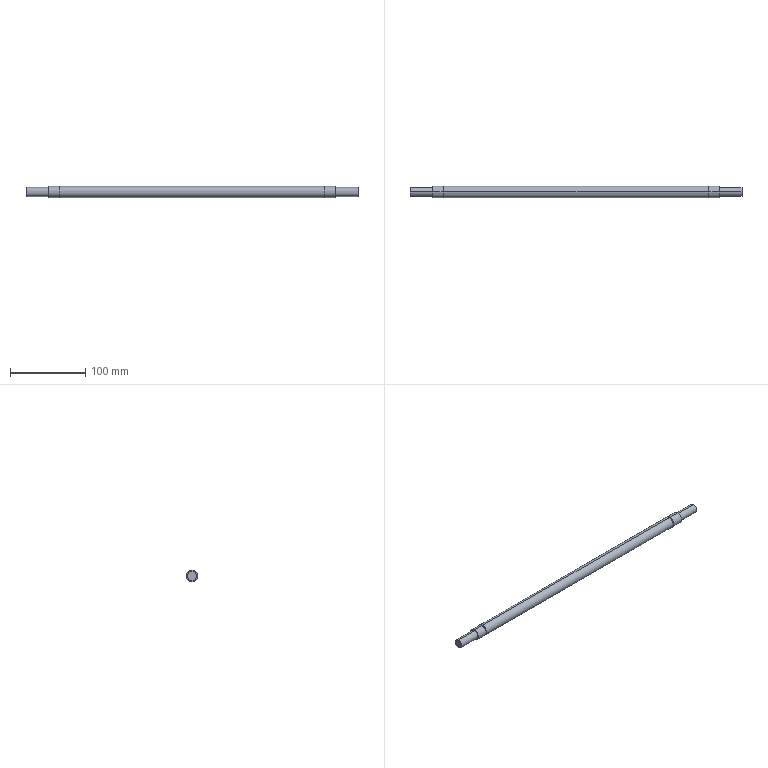Component | SolidWorks | 01-09MarkingMachineIdlerRollerAxis-2 | 1 solid | 22 faces | box 440 x 15 x 15 mm | volume 73902 mm3 | cylinder 14 | plane 8 | commonest cylinder face diameters 15 x6 12 x4 14.3 x4 | material A3 Steel
build123d program:
from build123d import *


with BuildPart() as part:
    # Sketch1 → Revolve1 (revolve)
    with BuildSketch(Plane.XY, mode=Mode.PRIVATE) as revolve1_sk:
        Polygon((-220, 0), (-220, 6), (-190, 6), (-190, 7.5), (-176.1, 7.5), (-176.1, 7.15), (-175, 7.15), (-175, 7.5), (175, 7.5), (175, 7.15), (176.1, 7.15), (176.1, 7.5), (190, 7.5), (190, 6), (220, 6), (220, 0), align=None)
    revolve(revolve1_sk.sketch.rotate(Axis((-253.202, 0, 0), (1, 0, 0)), 90), axis=Axis((-253.202, 0, 0), (1, 0, 0)))


solid = part.part

# Placed as in the assembly
solid = solid.moved(Location((-256.91, 57.41, 27.5), (0, 0, 0)))
STEP:
#1=COLOUR_RGB('',0.7922,0.8196,0.9333);
#2=FILL_AREA_STYLE_COLOUR('',#1);
#3=FILL_AREA_STYLE('',(#2));
#4=SURFACE_STYLE_FILL_AREA(#3);
#5=SURFACE_SIDE_STYLE('',(#4));
#6=SURFACE_STYLE_USAGE(.BOTH.,#5);
#7=PRESENTATION_STYLE_ASSIGNMENT((#6));
#8=CARTESIAN_POINT('',(-17.595,2.26,1.319));
#9=VERTEX_POINT('',#8);
#10=CARTESIAN_POINT('',(-17.595,2.26,0.8465));
#11=VERTEX_POINT('',#10);
#12=CARTESIAN_POINT('',(-17.595,2.26,1.083));
#13=DIRECTION('',(-1.,0.,0.));
#14=DIRECTION('',(0.,0.,1.));
#15=AXIS2_PLACEMENT_3D('',#12,#13,#14);
#16=CIRCLE('',#15,0.2362);
#17=EDGE_CURVE('',#9,#11,#16,.T.);
#18=ORIENTED_EDGE('',*,*,#17,.T.);
#19=CARTESIAN_POINT('',(-18.776,2.26,0.8465));
#20=VERTEX_POINT('',#19);
#21=CARTESIAN_POINT('',(-20.083,2.26,0.8465));
#22=DIRECTION('',(-1.,0.,0.));
#23=VECTOR('',#22,39.37);
#24=LINE('',#21,#23);
#25=EDGE_CURVE('',#11,#20,#24,.T.);
#26=ORIENTED_EDGE('',*,*,#25,.T.);
#27=CARTESIAN_POINT('',(-18.776,2.26,1.319));
#28=VERTEX_POINT('',#27);
#29=CARTESIAN_POINT('',(-18.776,2.26,1.083));
#30=DIRECTION('',(-1.,0.,0.));
#31=DIRECTION('',(0.,0.,1.));
#32=AXIS2_PLACEMENT_3D('',#29,#30,#31);
#33=CIRCLE('',#32,0.2362);
#34=EDGE_CURVE('',#28,#20,#33,.T.);
#35=ORIENTED_EDGE('',*,*,#34,.F.);
#36=CARTESIAN_POINT('',(-20.083,2.26,1.319));
#37=DIRECTION('',(-1.,0.,0.));
#38=VECTOR('',#37,39.37);
#39=LINE('',#36,#38);
#40=EDGE_CURVE('',#9,#28,#39,.T.);
#41=ORIENTED_EDGE('',*,*,#40,.F.);
#42=EDGE_LOOP('',(#18,#26,#35,#41));
#43=FACE_OUTER_BOUND('',#42,.T.);
#44=CARTESIAN_POINT('',(-20.083,2.26,1.083));
#45=DIRECTION('',(-1.,0.,0.));
#46=DIRECTION('',(0.,0.,1.));
#47=AXIS2_PLACEMENT_3D('',#44,#45,#46);
#48=CYLINDRICAL_SURFACE('',#47,0.2362);
#49=ADVANCED_FACE('',(#43),#48,.T.);
#50=CARTESIAN_POINT('',(-17.048,2.26,1.378));
#51=VERTEX_POINT('',#50);
#52=CARTESIAN_POINT('',(-17.048,2.26,0.7874));
#53=VERTEX_POINT('',#52);
#54=CARTESIAN_POINT('',(-17.048,2.26,1.083));
#55=DIRECTION('',(-1.,0.,0.));
#56=DIRECTION('',(0.,0.,1.));
#57=AXIS2_PLACEMENT_3D('',#54,#55,#56);
#58=CIRCLE('',#57,0.2953);
#59=EDGE_CURVE('',#51,#53,#58,.T.);
#60=ORIENTED_EDGE('',*,*,#59,.T.);
#61=CARTESIAN_POINT('',(-17.595,2.26,0.7874));
#62=VERTEX_POINT('',#61);
#63=CARTESIAN_POINT('',(-20.083,2.26,0.7874));
#64=DIRECTION('',(-1.,0.,0.));
#65=VECTOR('',#64,39.37);
#66=LINE('',#63,#65);
#67=EDGE_CURVE('',#53,#62,#66,.T.);
#68=ORIENTED_EDGE('',*,*,#67,.T.);
#69=CARTESIAN_POINT('',(-17.595,2.26,1.378));
#70=VERTEX_POINT('',#69);
#71=CARTESIAN_POINT('',(-17.595,2.26,1.083));
#72=DIRECTION('',(-1.,0.,0.));
#73=DIRECTION('',(0.,0.,1.));
#74=AXIS2_PLACEMENT_3D('',#71,#72,#73);
#75=CIRCLE('',#74,0.2953);
#76=EDGE_CURVE('',#70,#62,#75,.T.);
#77=ORIENTED_EDGE('',*,*,#76,.F.);
#78=CARTESIAN_POINT('',(-20.083,2.26,1.378));
#79=DIRECTION('',(-1.,0.,0.));
#80=VECTOR('',#79,39.37);
#81=LINE('',#78,#80);
#82=EDGE_CURVE('',#51,#70,#81,.T.);
#83=ORIENTED_EDGE('',*,*,#82,.F.);
#84=EDGE_LOOP('',(#60,#68,#77,#83));
#85=FACE_OUTER_BOUND('',#84,.T.);
#86=CARTESIAN_POINT('',(-20.083,2.26,1.083));
#87=DIRECTION('',(-1.,0.,0.));
#88=DIRECTION('',(0.,0.,1.));
#89=AXIS2_PLACEMENT_3D('',#86,#87,#88);
#90=CYLINDRICAL_SURFACE('',#89,0.2953);
#91=ADVANCED_FACE('',(#85),#90,.T.);
#92=CARTESIAN_POINT('',(-17.004,2.26,1.364));
#93=VERTEX_POINT('',#92);
#94=CARTESIAN_POINT('',(-17.004,2.26,0.8012));
#95=VERTEX_POINT('',#94);
#96=CARTESIAN_POINT('',(-17.004,2.26,1.083));
#97=DIRECTION('',(-1.,0.,0.));
#98=DIRECTION('',(0.,0.,1.));
#99=AXIS2_PLACEMENT_3D('',#96,#97,#98);
#100=CIRCLE('',#99,0.2815);
#101=EDGE_CURVE('',#93,#95,#100,.T.);
#102=ORIENTED_EDGE('',*,*,#101,.T.);
#103=CARTESIAN_POINT('',(-17.048,2.26,0.8012));
#104=VERTEX_POINT('',#103);
#105=CARTESIAN_POINT('',(-20.083,2.26,0.8012));
#106=DIRECTION('',(-1.,0.,0.));
#107=VECTOR('',#106,39.37);
#108=LINE('',#105,#107);
#109=EDGE_CURVE('',#95,#104,#108,.T.);
#110=ORIENTED_EDGE('',*,*,#109,.T.);
#111=CARTESIAN_POINT('',(-17.048,2.26,1.364));
#112=VERTEX_POINT('',#111);
#113=CARTESIAN_POINT('',(-17.048,2.26,1.083));
#114=DIRECTION('',(-1.,0.,0.));
#115=DIRECTION('',(0.,0.,1.));
#116=AXIS2_PLACEMENT_3D('',#113,#114,#115);
#117=CIRCLE('',#116,0.2815);
#118=EDGE_CURVE('',#112,#104,#117,.T.);
#119=ORIENTED_EDGE('',*,*,#118,.F.);
#120=CARTESIAN_POINT('',(-20.083,2.26,1.364));
#121=DIRECTION('',(-1.,0.,0.));
#122=VECTOR('',#121,39.37);
#123=LINE('',#120,#122);
#124=EDGE_CURVE('',#93,#112,#123,.T.);
#125=ORIENTED_EDGE('',*,*,#124,.F.);
#126=EDGE_LOOP('',(#102,#110,#119,#125));
#127=FACE_OUTER_BOUND('',#126,.T.);
#128=CARTESIAN_POINT('',(-20.083,2.26,1.083));
#129=DIRECTION('',(-1.,0.,0.));
#130=DIRECTION('',(0.,0.,1.));
#131=AXIS2_PLACEMENT_3D('',#128,#129,#130);
#132=CYLINDRICAL_SURFACE('',#131,0.2815);
#133=ADVANCED_FACE('',(#127),#132,.T.);
#134=CARTESIAN_POINT('',(-3.225,2.26,1.378));
#135=VERTEX_POINT('',#134);
#136=CARTESIAN_POINT('',(-3.225,2.26,0.7874));
#137=VERTEX_POINT('',#136);
#138=CARTESIAN_POINT('',(-3.225,2.26,1.083));
#139=DIRECTION('',(-1.,0.,0.));
#140=DIRECTION('',(0.,0.,1.));
#141=AXIS2_PLACEMENT_3D('',#138,#139,#140);
#142=CIRCLE('',#141,0.2953);
#143=EDGE_CURVE('',#135,#137,#142,.T.);
#144=ORIENTED_EDGE('',*,*,#143,.T.);
#145=CARTESIAN_POINT('',(-17.004,2.26,0.7874));
#146=VERTEX_POINT('',#145);
#147=CARTESIAN_POINT('',(-20.083,2.26,0.7874));
#148=DIRECTION('',(-1.,0.,0.));
#149=VECTOR('',#148,39.37);
#150=LINE('',#147,#149);
#151=EDGE_CURVE('',#137,#146,#150,.T.);
#152=ORIENTED_EDGE('',*,*,#151,.T.);
#153=CARTESIAN_POINT('',(-17.004,2.26,1.378));
#154=VERTEX_POINT('',#153);
#155=CARTESIAN_POINT('',(-17.004,2.26,1.083));
#156=DIRECTION('',(-1.,0.,0.));
#157=DIRECTION('',(0.,0.,1.));
#158=AXIS2_PLACEMENT_3D('',#155,#156,#157);
#159=CIRCLE('',#158,0.2953);
#160=EDGE_CURVE('',#154,#146,#159,.T.);
#161=ORIENTED_EDGE('',*,*,#160,.F.);
#162=CARTESIAN_POINT('',(-20.083,2.26,1.378));
#163=DIRECTION('',(-1.,0.,0.));
#164=VECTOR('',#163,39.37);
#165=LINE('',#162,#164);
#166=EDGE_CURVE('',#135,#154,#165,.T.);
#167=ORIENTED_EDGE('',*,*,#166,.F.);
#168=EDGE_LOOP('',(#144,#152,#161,#167));
#169=FACE_OUTER_BOUND('',#168,.T.);
#170=CARTESIAN_POINT('',(-20.083,2.26,1.083));
#171=DIRECTION('',(-1.,0.,0.));
#172=DIRECTION('',(0.,0.,1.));
#173=AXIS2_PLACEMENT_3D('',#170,#171,#172);
#174=CYLINDRICAL_SURFACE('',#173,0.2953);
#175=ADVANCED_FACE('',(#169),#174,.T.);
#176=CARTESIAN_POINT('',(-3.182,2.26,1.364));
#177=VERTEX_POINT('',#176);
#178=CARTESIAN_POINT('',(-3.182,2.26,0.8012));
#179=VERTEX_POINT('',#178);
#180=CARTESIAN_POINT('',(-3.182,2.26,1.083));
#181=DIRECTION('',(-1.,0.,0.));
#182=DIRECTION('',(0.,0.,1.));
#183=AXIS2_PLACEMENT_3D('',#180,#181,#182);
#184=CIRCLE('',#183,0.2815);
#185=EDGE_CURVE('',#177,#179,#184,.T.);
#186=ORIENTED_EDGE('',*,*,#185,.T.);
#187=CARTESIAN_POINT('',(-3.225,2.26,0.8012));
#188=VERTEX_POINT('',#187);
#189=CARTESIAN_POINT('',(-20.083,2.26,0.8012));
#190=DIRECTION('',(-1.,0.,0.));
#191=VECTOR('',#190,39.37);
#192=LINE('',#189,#191);
#193=EDGE_CURVE('',#179,#188,#192,.T.);
#194=ORIENTED_EDGE('',*,*,#193,.T.);
#195=CARTESIAN_POINT('',(-3.225,2.26,1.364));
#196=VERTEX_POINT('',#195);
#197=CARTESIAN_POINT('',(-3.225,2.26,1.083));
#198=DIRECTION('',(-1.,0.,0.));
#199=DIRECTION('',(0.,0.,1.));
#200=AXIS2_PLACEMENT_3D('',#197,#198,#199);
#201=CIRCLE('',#200,0.2815);
#202=EDGE_CURVE('',#196,#188,#201,.T.);
#203=ORIENTED_EDGE('',*,*,#202,.F.);
#204=CARTESIAN_POINT('',(-20.083,2.26,1.364));
#205=DIRECTION('',(-1.,0.,0.));
#206=VECTOR('',#205,39.37);
#207=LINE('',#204,#206);
#208=EDGE_CURVE('',#177,#196,#207,.T.);
#209=ORIENTED_EDGE('',*,*,#208,.F.);
#210=EDGE_LOOP('',(#186,#194,#203,#209));
#211=FACE_OUTER_BOUND('',#210,.T.);
#212=CARTESIAN_POINT('',(-20.083,2.26,1.083));
#213=DIRECTION('',(-1.,0.,0.));
#214=DIRECTION('',(0.,0.,1.));
#215=AXIS2_PLACEMENT_3D('',#212,#213,#214);
#216=CYLINDRICAL_SURFACE('',#215,0.2815);
#217=ADVANCED_FACE('',(#211),#216,.T.);
#218=CARTESIAN_POINT('',(-2.634,2.26,1.378));
#219=VERTEX_POINT('',#218);
#220=CARTESIAN_POINT('',(-2.634,2.26,0.7874));
#221=VERTEX_POINT('',#220);
#222=CARTESIAN_POINT('',(-2.634,2.26,1.083));
#223=DIRECTION('',(-1.,0.,0.));
#224=DIRECTION('',(0.,0.,1.));
#225=AXIS2_PLACEMENT_3D('',#222,#223,#224);
#226=CIRCLE('',#225,0.2953);
#227=EDGE_CURVE('',#219,#221,#226,.T.);
#228=ORIENTED_EDGE('',*,*,#227,.T.);
#229=CARTESIAN_POINT('',(-3.182,2.26,0.7874));
#230=VERTEX_POINT('',#229);
#231=CARTESIAN_POINT('',(-20.083,2.26,0.7874));
#232=DIRECTION('',(-1.,0.,0.));
#233=VECTOR('',#232,39.37);
#234=LINE('',#231,#233);
#235=EDGE_CURVE('',#221,#230,#234,.T.);
#236=ORIENTED_EDGE('',*,*,#235,.T.);
#237=CARTESIAN_POINT('',(-3.182,2.26,1.378));
#238=VERTEX_POINT('',#237);
#239=CARTESIAN_POINT('',(-3.182,2.26,1.083));
#240=DIRECTION('',(-1.,0.,0.));
#241=DIRECTION('',(0.,0.,1.));
#242=AXIS2_PLACEMENT_3D('',#239,#240,#241);
#243=CIRCLE('',#242,0.2953);
#244=EDGE_CURVE('',#238,#230,#243,.T.);
#245=ORIENTED_EDGE('',*,*,#244,.F.);
#246=CARTESIAN_POINT('',(-20.083,2.26,1.378));
#247=DIRECTION('',(-1.,0.,0.));
#248=VECTOR('',#247,39.37);
#249=LINE('',#246,#248);
#250=EDGE_CURVE('',#219,#238,#249,.T.);
#251=ORIENTED_EDGE('',*,*,#250,.F.);
#252=EDGE_LOOP('',(#228,#236,#245,#251));
#253=FACE_OUTER_BOUND('',#252,.T.);
#254=CARTESIAN_POINT('',(-20.083,2.26,1.083));
#255=DIRECTION('',(-1.,0.,0.));
#256=DIRECTION('',(0.,0.,1.));
#257=AXIS2_PLACEMENT_3D('',#254,#255,#256);
#258=CYLINDRICAL_SURFACE('',#257,0.2953);
#259=ADVANCED_FACE('',(#253),#258,.T.);
#260=CARTESIAN_POINT('',(-1.453,2.26,1.319));
#261=VERTEX_POINT('',#260);
#262=CARTESIAN_POINT('',(-1.453,2.26,0.8465));
#263=VERTEX_POINT('',#262);
#264=CARTESIAN_POINT('',(-1.453,2.26,1.083));
#265=DIRECTION('',(-1.,0.,0.));
#266=DIRECTION('',(0.,0.,1.));
#267=AXIS2_PLACEMENT_3D('',#264,#265,#266);
#268=CIRCLE('',#267,0.2362);
#269=EDGE_CURVE('',#261,#263,#268,.T.);
#270=ORIENTED_EDGE('',*,*,#269,.T.);
#271=CARTESIAN_POINT('',(-2.634,2.26,0.8465));
#272=VERTEX_POINT('',#271);
#273=CARTESIAN_POINT('',(-20.083,2.26,0.8465));
#274=DIRECTION('',(-1.,0.,0.));
#275=VECTOR('',#274,39.37);
#276=LINE('',#273,#275);
#277=EDGE_CURVE('',#263,#272,#276,.T.);
#278=ORIENTED_EDGE('',*,*,#277,.T.);
#279=CARTESIAN_POINT('',(-2.634,2.26,1.319));
#280=VERTEX_POINT('',#279);
#281=CARTESIAN_POINT('',(-2.634,2.26,1.083));
#282=DIRECTION('',(-1.,0.,0.));
#283=DIRECTION('',(0.,0.,1.));
#284=AXIS2_PLACEMENT_3D('',#281,#282,#283);
#285=CIRCLE('',#284,0.2362);
#286=EDGE_CURVE('',#280,#272,#285,.T.);
#287=ORIENTED_EDGE('',*,*,#286,.F.);
#288=CARTESIAN_POINT('',(-20.083,2.26,1.319));
#289=DIRECTION('',(-1.,0.,0.));
#290=VECTOR('',#289,39.37);
#291=LINE('',#288,#290);
#292=EDGE_CURVE('',#261,#280,#291,.T.);
#293=ORIENTED_EDGE('',*,*,#292,.F.);
#294=EDGE_LOOP('',(#270,#278,#287,#293));
#295=FACE_OUTER_BOUND('',#294,.T.);
#296=CARTESIAN_POINT('',(-20.083,2.26,1.083));
#297=DIRECTION('',(-1.,0.,0.));
#298=DIRECTION('',(0.,0.,1.));
#299=AXIS2_PLACEMENT_3D('',#296,#297,#298);
#300=CYLINDRICAL_SURFACE('',#299,0.2362);
#301=ADVANCED_FACE('',(#295),#300,.T.);
#302=ORIENTED_EDGE('',*,*,#269,.F.);
#303=CARTESIAN_POINT('',(-1.453,2.26,1.083));
#304=DIRECTION('',(-1.,0.,0.));
#305=DIRECTION('',(0.,0.,1.));
#306=AXIS2_PLACEMENT_3D('',#303,#304,#305);
#307=CIRCLE('',#306,0.2362);
#308=EDGE_CURVE('',#263,#261,#307,.T.);
#309=ORIENTED_EDGE('',*,*,#308,.F.);
#310=EDGE_LOOP('',(#302,#309));
#311=FACE_OUTER_BOUND('',#310,.T.);
#312=CARTESIAN_POINT('',(-1.453,2.26,1.083));
#313=DIRECTION('',(-1.,0.,0.));
#314=DIRECTION('',(0.,0.,1.));
#315=AXIS2_PLACEMENT_3D('',#312,#313,#314);
#316=PLANE('',#315);
#317=ADVANCED_FACE('',(#311),#316,.F.);
#318=ORIENTED_EDGE('',*,*,#277,.F.);
#319=ORIENTED_EDGE('',*,*,#308,.T.);
#320=ORIENTED_EDGE('',*,*,#292,.T.);
#321=CARTESIAN_POINT('',(-2.634,2.26,1.083));
#322=DIRECTION('',(-1.,0.,0.));
#323=DIRECTION('',(0.,0.,1.));
#324=AXIS2_PLACEMENT_3D('',#321,#322,#323);
#325=CIRCLE('',#324,0.2362);
#326=EDGE_CURVE('',#272,#280,#325,.T.);
#327=ORIENTED_EDGE('',*,*,#326,.F.);
#328=EDGE_LOOP('',(#318,#319,#320,#327));
#329=FACE_OUTER_BOUND('',#328,.T.);
#330=CARTESIAN_POINT('',(-20.083,2.26,1.083));
#331=DIRECTION('',(-1.,0.,0.));
#332=DIRECTION('',(0.,0.,1.));
#333=AXIS2_PLACEMENT_3D('',#330,#331,#332);
#334=CYLINDRICAL_SURFACE('',#333,0.2362);
#335=ADVANCED_FACE('',(#329),#334,.T.);
#336=ORIENTED_EDGE('',*,*,#227,.F.);
#337=CARTESIAN_POINT('',(-2.634,2.26,1.083));
#338=DIRECTION('',(-1.,0.,0.));
#339=DIRECTION('',(0.,0.,1.));
#340=AXIS2_PLACEMENT_3D('',#337,#338,#339);
#341=CIRCLE('',#340,0.2953);
#342=EDGE_CURVE('',#221,#219,#341,.T.);
#343=ORIENTED_EDGE('',*,*,#342,.F.);
#344=EDGE_LOOP('',(#336,#343));
#345=FACE_OUTER_BOUND('',#344,.T.);
#346=ORIENTED_EDGE('',*,*,#286,.T.);
#347=ORIENTED_EDGE('',*,*,#326,.T.);
#348=EDGE_LOOP('',(#346,#347));
#349=FACE_BOUND('',#348,.T.);
#350=CARTESIAN_POINT('',(-2.634,2.496,1.083));
#351=DIRECTION('',(-1.,0.,0.));
#352=DIRECTION('',(0.,0.,1.));
#353=AXIS2_PLACEMENT_3D('',#350,#351,#352);
#354=PLANE('',#353);
#355=ADVANCED_FACE('',(#345,#349),#354,.F.);
#356=ORIENTED_EDGE('',*,*,#235,.F.);
#357=ORIENTED_EDGE('',*,*,#342,.T.);
#358=ORIENTED_EDGE('',*,*,#250,.T.);
#359=CARTESIAN_POINT('',(-3.182,2.26,1.083));
#360=DIRECTION('',(-1.,0.,0.));
#361=DIRECTION('',(0.,0.,1.));
#362=AXIS2_PLACEMENT_3D('',#359,#360,#361);
#363=CIRCLE('',#362,0.2953);
#364=EDGE_CURVE('',#230,#238,#363,.T.);
#365=ORIENTED_EDGE('',*,*,#364,.F.);
#366=EDGE_LOOP('',(#356,#357,#358,#365));
#367=FACE_OUTER_BOUND('',#366,.T.);
#368=CARTESIAN_POINT('',(-20.083,2.26,1.083));
#369=DIRECTION('',(-1.,0.,0.));
#370=DIRECTION('',(0.,0.,1.));
#371=AXIS2_PLACEMENT_3D('',#368,#369,#370);
#372=CYLINDRICAL_SURFACE('',#371,0.2953);
#373=ADVANCED_FACE('',(#367),#372,.T.);
#374=ORIENTED_EDGE('',*,*,#185,.F.);
#375=CARTESIAN_POINT('',(-3.182,2.26,1.083));
#376=DIRECTION('',(-1.,0.,0.));
#377=DIRECTION('',(0.,0.,1.));
#378=AXIS2_PLACEMENT_3D('',#375,#376,#377);
#379=CIRCLE('',#378,0.2815);
#380=EDGE_CURVE('',#179,#177,#379,.T.);
#381=ORIENTED_EDGE('',*,*,#380,.F.);
#382=EDGE_LOOP('',(#374,#381));
#383=FACE_BOUND('',#382,.T.);
#384=ORIENTED_EDGE('',*,*,#244,.T.);
#385=ORIENTED_EDGE('',*,*,#364,.T.);
#386=EDGE_LOOP('',(#384,#385));
#387=FACE_OUTER_BOUND('',#386,.T.);
#388=CARTESIAN_POINT('',(-3.182,2.556,1.083));
#389=DIRECTION('',(1.,0.,0.));
#390=DIRECTION('',(0.,0.,-1.));
#391=AXIS2_PLACEMENT_3D('',#388,#389,#390);
#392=PLANE('',#391);
#393=ADVANCED_FACE('',(#383,#387),#392,.F.);
#394=ORIENTED_EDGE('',*,*,#193,.F.);
#395=ORIENTED_EDGE('',*,*,#380,.T.);
#396=ORIENTED_EDGE('',*,*,#208,.T.);
#397=CARTESIAN_POINT('',(-3.225,2.26,1.083));
#398=DIRECTION('',(-1.,0.,0.));
#399=DIRECTION('',(0.,0.,1.));
#400=AXIS2_PLACEMENT_3D('',#397,#398,#399);
#401=CIRCLE('',#400,0.2815);
#402=EDGE_CURVE('',#188,#196,#401,.T.);
#403=ORIENTED_EDGE('',*,*,#402,.F.);
#404=EDGE_LOOP('',(#394,#395,#396,#403));
#405=FACE_OUTER_BOUND('',#404,.T.);
#406=CARTESIAN_POINT('',(-20.083,2.26,1.083));
#407=DIRECTION('',(-1.,0.,0.));
#408=DIRECTION('',(0.,0.,1.));
#409=AXIS2_PLACEMENT_3D('',#406,#407,#408);
#410=CYLINDRICAL_SURFACE('',#409,0.2815);
#411=ADVANCED_FACE('',(#405),#410,.T.);
#412=ORIENTED_EDGE('',*,*,#143,.F.);
#413=CARTESIAN_POINT('',(-3.225,2.26,1.083));
#414=DIRECTION('',(-1.,0.,0.));
#415=DIRECTION('',(0.,0.,1.));
#416=AXIS2_PLACEMENT_3D('',#413,#414,#415);
#417=CIRCLE('',#416,0.2953);
#418=EDGE_CURVE('',#137,#135,#417,.T.);
#419=ORIENTED_EDGE('',*,*,#418,.F.);
#420=EDGE_LOOP('',(#412,#419));
#421=FACE_OUTER_BOUND('',#420,.T.);
#422=ORIENTED_EDGE('',*,*,#202,.T.);
#423=ORIENTED_EDGE('',*,*,#402,.T.);
#424=EDGE_LOOP('',(#422,#423));
#425=FACE_BOUND('',#424,.T.);
#426=CARTESIAN_POINT('',(-3.225,2.542,1.083));
#427=DIRECTION('',(-1.,0.,0.));
#428=DIRECTION('',(0.,0.,1.));
#429=AXIS2_PLACEMENT_3D('',#426,#427,#428);
#430=PLANE('',#429);
#431=ADVANCED_FACE('',(#421,#425),#430,.F.);
#432=ORIENTED_EDGE('',*,*,#151,.F.);
#433=ORIENTED_EDGE('',*,*,#418,.T.);
#434=ORIENTED_EDGE('',*,*,#166,.T.);
#435=CARTESIAN_POINT('',(-17.004,2.26,1.083));
#436=DIRECTION('',(-1.,0.,0.));
#437=DIRECTION('',(0.,0.,1.));
#438=AXIS2_PLACEMENT_3D('',#435,#436,#437);
#439=CIRCLE('',#438,0.2953);
#440=EDGE_CURVE('',#146,#154,#439,.T.);
#441=ORIENTED_EDGE('',*,*,#440,.F.);
#442=EDGE_LOOP('',(#432,#433,#434,#441));
#443=FACE_OUTER_BOUND('',#442,.T.);
#444=CARTESIAN_POINT('',(-20.083,2.26,1.083));
#445=DIRECTION('',(-1.,0.,0.));
#446=DIRECTION('',(0.,0.,1.));
#447=AXIS2_PLACEMENT_3D('',#444,#445,#446);
#448=CYLINDRICAL_SURFACE('',#447,0.2953);
#449=ADVANCED_FACE('',(#443),#448,.T.);
#450=ORIENTED_EDGE('',*,*,#101,.F.);
#451=CARTESIAN_POINT('',(-17.004,2.26,1.083));
#452=DIRECTION('',(-1.,0.,0.));
#453=DIRECTION('',(0.,0.,1.));
#454=AXIS2_PLACEMENT_3D('',#451,#452,#453);
#455=CIRCLE('',#454,0.2815);
#456=EDGE_CURVE('',#95,#93,#455,.T.);
#457=ORIENTED_EDGE('',*,*,#456,.F.);
#458=EDGE_LOOP('',(#450,#457));
#459=FACE_BOUND('',#458,.T.);
#460=ORIENTED_EDGE('',*,*,#160,.T.);
#461=ORIENTED_EDGE('',*,*,#440,.T.);
#462=EDGE_LOOP('',(#460,#461));
#463=FACE_OUTER_BOUND('',#462,.T.);
#464=CARTESIAN_POINT('',(-17.004,2.542,1.083));
#465=DIRECTION('',(1.,0.,0.));
#466=DIRECTION('',(0.,0.,-1.));
#467=AXIS2_PLACEMENT_3D('',#464,#465,#466);
#468=PLANE('',#467);
#469=ADVANCED_FACE('',(#459,#463),#468,.F.);
#470=ORIENTED_EDGE('',*,*,#109,.F.);
#471=ORIENTED_EDGE('',*,*,#456,.T.);
#472=ORIENTED_EDGE('',*,*,#124,.T.);
#473=CARTESIAN_POINT('',(-17.048,2.26,1.083));
#474=DIRECTION('',(-1.,0.,0.));
#475=DIRECTION('',(0.,0.,1.));
#476=AXIS2_PLACEMENT_3D('',#473,#474,#475);
#477=CIRCLE('',#476,0.2815);
#478=EDGE_CURVE('',#104,#112,#477,.T.);
#479=ORIENTED_EDGE('',*,*,#478,.F.);
#480=EDGE_LOOP('',(#470,#471,#472,#479));
#481=FACE_OUTER_BOUND('',#480,.T.);
#482=CARTESIAN_POINT('',(-20.083,2.26,1.083));
#483=DIRECTION('',(-1.,0.,0.));
#484=DIRECTION('',(0.,0.,1.));
#485=AXIS2_PLACEMENT_3D('',#482,#483,#484);
#486=CYLINDRICAL_SURFACE('',#485,0.2815);
#487=ADVANCED_FACE('',(#481),#486,.T.);
#488=ORIENTED_EDGE('',*,*,#59,.F.);
#489=CARTESIAN_POINT('',(-17.048,2.26,1.083));
#490=DIRECTION('',(-1.,0.,0.));
#491=DIRECTION('',(0.,0.,1.));
#492=AXIS2_PLACEMENT_3D('',#489,#490,#491);
#493=CIRCLE('',#492,0.2953);
#494=EDGE_CURVE('',#53,#51,#493,.T.);
#495=ORIENTED_EDGE('',*,*,#494,.F.);
#496=EDGE_LOOP('',(#488,#495));
#497=FACE_OUTER_BOUND('',#496,.T.);
#498=ORIENTED_EDGE('',*,*,#118,.T.);
#499=ORIENTED_EDGE('',*,*,#478,.T.);
#500=EDGE_LOOP('',(#498,#499));
#501=FACE_BOUND('',#500,.T.);
#502=CARTESIAN_POINT('',(-17.048,2.556,1.083));
#503=DIRECTION('',(-1.,0.,0.));
#504=DIRECTION('',(0.,0.,1.));
#505=AXIS2_PLACEMENT_3D('',#502,#503,#504);
#506=PLANE('',#505);
#507=ADVANCED_FACE('',(#497,#501),#506,.F.);
#508=ORIENTED_EDGE('',*,*,#67,.F.);
#509=ORIENTED_EDGE('',*,*,#494,.T.);
#510=ORIENTED_EDGE('',*,*,#82,.T.);
#511=CARTESIAN_POINT('',(-17.595,2.26,1.083));
#512=DIRECTION('',(-1.,0.,0.));
#513=DIRECTION('',(0.,0.,1.));
#514=AXIS2_PLACEMENT_3D('',#511,#512,#513);
#515=CIRCLE('',#514,0.2953);
#516=EDGE_CURVE('',#62,#70,#515,.T.);
#517=ORIENTED_EDGE('',*,*,#516,.F.);
#518=EDGE_LOOP('',(#508,#509,#510,#517));
#519=FACE_OUTER_BOUND('',#518,.T.);
#520=CARTESIAN_POINT('',(-20.083,2.26,1.083));
#521=DIRECTION('',(-1.,0.,0.));
#522=DIRECTION('',(0.,0.,1.));
#523=AXIS2_PLACEMENT_3D('',#520,#521,#522);
#524=CYLINDRICAL_SURFACE('',#523,0.2953);
#525=ADVANCED_FACE('',(#519),#524,.T.);
#526=ORIENTED_EDGE('',*,*,#17,.F.);
#527=CARTESIAN_POINT('',(-17.595,2.26,1.083));
#528=DIRECTION('',(-1.,0.,0.));
#529=DIRECTION('',(0.,0.,1.));
#530=AXIS2_PLACEMENT_3D('',#527,#528,#529);
#531=CIRCLE('',#530,0.2362);
#532=EDGE_CURVE('',#11,#9,#531,.T.);
#533=ORIENTED_EDGE('',*,*,#532,.F.);
#534=EDGE_LOOP('',(#526,#533));
#535=FACE_BOUND('',#534,.T.);
#536=ORIENTED_EDGE('',*,*,#76,.T.);
#537=ORIENTED_EDGE('',*,*,#516,.T.);
#538=EDGE_LOOP('',(#536,#537));
#539=FACE_OUTER_BOUND('',#538,.T.);
#540=CARTESIAN_POINT('',(-17.595,2.496,1.083));
#541=DIRECTION('',(1.,0.,0.));
#542=DIRECTION('',(0.,0.,-1.));
#543=AXIS2_PLACEMENT_3D('',#540,#541,#542);
#544=PLANE('',#543);
#545=ADVANCED_FACE('',(#535,#539),#544,.F.);
#546=ORIENTED_EDGE('',*,*,#25,.F.);
#547=ORIENTED_EDGE('',*,*,#532,.T.);
#548=ORIENTED_EDGE('',*,*,#40,.T.);
#549=CARTESIAN_POINT('',(-18.776,2.26,1.083));
#550=DIRECTION('',(-1.,0.,0.));
#551=DIRECTION('',(0.,0.,1.));
#552=AXIS2_PLACEMENT_3D('',#549,#550,#551);
#553=CIRCLE('',#552,0.2362);
#554=EDGE_CURVE('',#20,#28,#553,.T.);
#555=ORIENTED_EDGE('',*,*,#554,.F.);
#556=EDGE_LOOP('',(#546,#547,#548,#555));
#557=FACE_OUTER_BOUND('',#556,.T.);
#558=CARTESIAN_POINT('',(-20.083,2.26,1.083));
#559=DIRECTION('',(-1.,0.,0.));
#560=DIRECTION('',(0.,0.,1.));
#561=AXIS2_PLACEMENT_3D('',#558,#559,#560);
#562=CYLINDRICAL_SURFACE('',#561,0.2362);
#563=ADVANCED_FACE('',(#557),#562,.T.);
#564=ORIENTED_EDGE('',*,*,#34,.T.);
#565=ORIENTED_EDGE('',*,*,#554,.T.);
#566=EDGE_LOOP('',(#564,#565));
#567=FACE_OUTER_BOUND('',#566,.T.);
#568=CARTESIAN_POINT('',(-18.776,2.26,1.083));
#569=DIRECTION('',(1.,0.,0.));
#570=DIRECTION('',(0.,0.,-1.));
#571=AXIS2_PLACEMENT_3D('',#568,#569,#570);
#572=PLANE('',#571);
#573=ADVANCED_FACE('',(#567),#572,.F.);
#574=CLOSED_SHELL('',(#49,#91,#133,#175,#217,#259,#301,#317,#335,#355,#373,#393,#411,#431,#449,#469,#487,#507,#525,#545,#563,#573));
#575=MANIFOLD_SOLID_BREP('',#574);
#576=STYLED_ITEM('',(#7),#575);
#577=PRESENTATION_LAYER_ASSIGNMENT('','',(#576));
#578=(LENGTH_UNIT()NAMED_UNIT(*)SI_UNIT($,.METRE.));
#579=LENGTH_MEASURE_WITH_UNIT(LENGTH_MEASURE(0.0254),#578);
#580=DIMENSIONAL_EXPONENTS(1.,0.,0.,0.,0.,0.,0.);
#581=(CONVERSION_BASED_UNIT('',#579)LENGTH_UNIT()NAMED_UNIT(#580));
#582=UNCERTAINTY_MEASURE_WITH_UNIT(LENGTH_MEASURE(0.00001),#581,'','');
#583=(NAMED_UNIT(*)PLANE_ANGLE_UNIT()SI_UNIT($,.RADIAN.));
#584=(NAMED_UNIT(*)SI_UNIT($,.STERADIAN.)SOLID_ANGLE_UNIT());
#585=(GEOMETRIC_REPRESENTATION_CONTEXT(3)GLOBAL_UNCERTAINTY_ASSIGNED_CONTEXT((#582))GLOBAL_UNIT_ASSIGNED_CONTEXT((#581,#583,#584))REPRESENTATION_CONTEXT('',''));
#586=MECHANICAL_DESIGN_GEOMETRIC_PRESENTATION_REPRESENTATION('',(#576),#585);
#587=CARTESIAN_POINT('',(0.,0.,0.));
#588=DIRECTION('',(0.,0.,1.));
#589=DIRECTION('',(1.,0.,0.));
#590=AXIS2_PLACEMENT_3D('',#587,#588,#589);
#591=(LENGTH_UNIT()NAMED_UNIT(*)SI_UNIT($,.METRE.));
#592=LENGTH_MEASURE_WITH_UNIT(LENGTH_MEASURE(0.0254),#591);
#593=DIMENSIONAL_EXPONENTS(1.,0.,0.,0.,0.,0.,0.);
#594=(CONVERSION_BASED_UNIT('',#592)LENGTH_UNIT()NAMED_UNIT(#593));
#595=UNCERTAINTY_MEASURE_WITH_UNIT(LENGTH_MEASURE(0.00001),#594,'','');
#596=(NAMED_UNIT(*)PLANE_ANGLE_UNIT()SI_UNIT($,.RADIAN.));
#597=(NAMED_UNIT(*)SI_UNIT($,.STERADIAN.)SOLID_ANGLE_UNIT());
#598=(GEOMETRIC_REPRESENTATION_CONTEXT(3)GLOBAL_UNCERTAINTY_ASSIGNED_CONTEXT((#595))GLOBAL_UNIT_ASSIGNED_CONTEXT((#594,#596,#597))REPRESENTATION_CONTEXT('',''));
#599=ADVANCED_BREP_SHAPE_REPRESENTATION('',(#575,#590),#598);